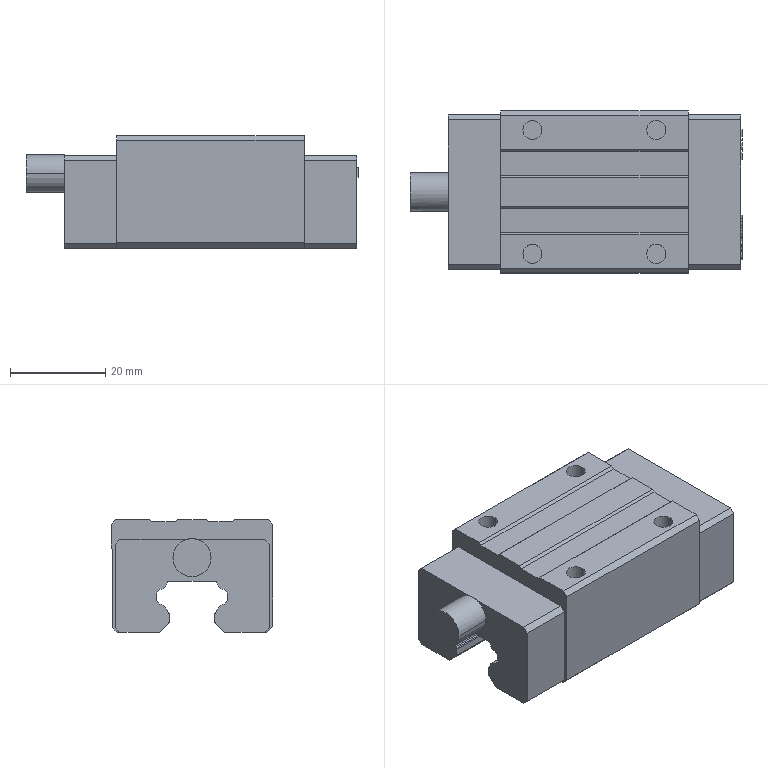Component | SolidWorks | SliderHIWINHGH15CA-C-1 | 1 solid | 420 faces | box 69.7 x 34 x 23.7 mm | volume 37448 mm3 | plane 291 | spline 107 | cylinder 22 | commonest cylinder face diameters 4 x8 0.8 x8 3.24 x4 8 x2